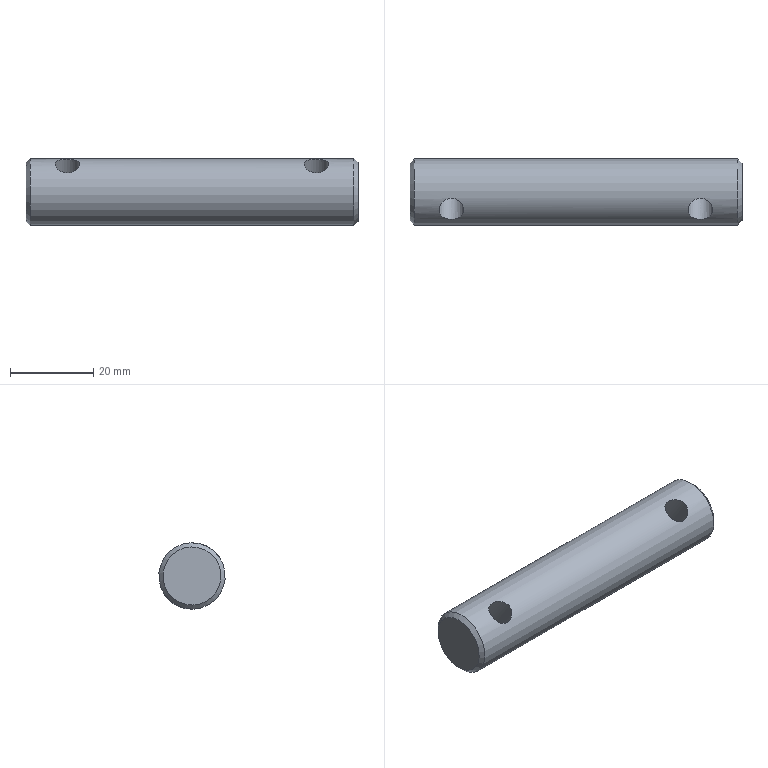Component | NX | KEY_2 | 1 solid | 7 faces | volume 15148 mm3 | cylinder 3 | plane 2 | cone 2 | commonest cylinder face diameters 6 x2 16 x1